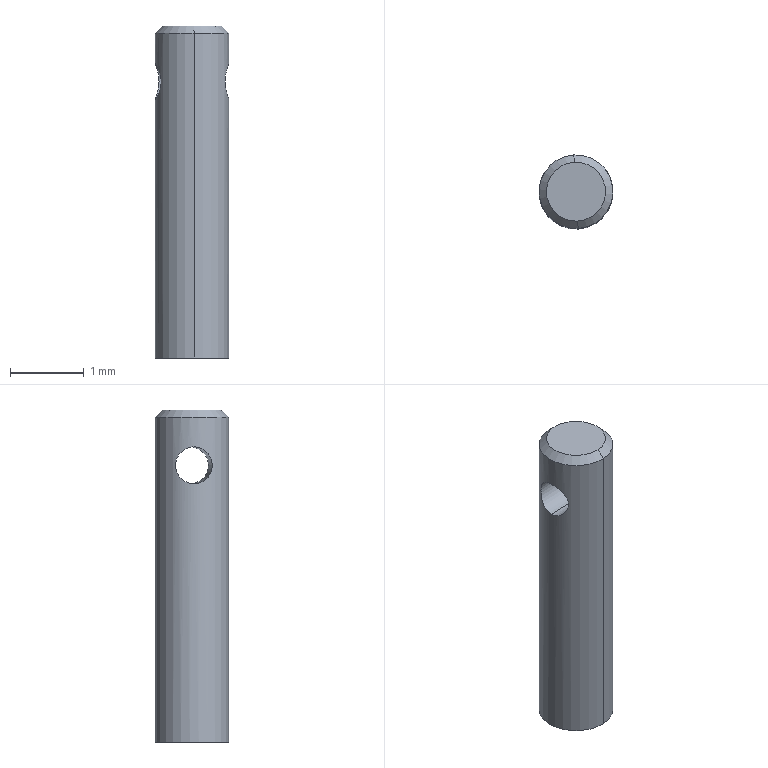Component | SolidWorks | Part25^Assembly1-2 | 1 solid | 8 faces | box 1 x 1 x 4.5 mm | volume 3 mm3 | cylinder 4 | cone 2 | plane 2 | commonest cylinder face diameters 0.5 x2 1 x2
STEP:
#1=COLOUR_RGB('',0.7922,0.8196,0.9333);
#2=FILL_AREA_STYLE_COLOUR('',#1);
#3=FILL_AREA_STYLE('',(#2));
#4=SURFACE_STYLE_FILL_AREA(#3);
#5=SURFACE_SIDE_STYLE('',(#4));
#6=SURFACE_STYLE_USAGE(.BOTH.,#5);
#7=PRESENTATION_STYLE_ASSIGNMENT((#6));
#8=CARTESIAN_POINT('',(0.368,-0.1104,0.3543));
#9=VERTEX_POINT('',#8);
#10=CARTESIAN_POINT('',(0.368,-0.1104,0.3346));
#11=VERTEX_POINT('',#10);
#12=CARTESIAN_POINT('',(0.368,-0.1104,0.3543));
#13=CARTESIAN_POINT('',(0.3682,-0.113,0.3543));
#14=CARTESIAN_POINT('',(0.3689,-0.1156,0.3532));
#15=CARTESIAN_POINT('',(0.3705,-0.1191,0.3496));
#16=CARTESIAN_POINT('',(0.3712,-0.1201,0.3471));
#17=CARTESIAN_POINT('',(0.3712,-0.1201,0.3419));
#18=CARTESIAN_POINT('',(0.3705,-0.1191,0.3393));
#19=CARTESIAN_POINT('',(0.3689,-0.1156,0.3357));
#20=CARTESIAN_POINT('',(0.3682,-0.1131,0.3346));
#21=CARTESIAN_POINT('',(0.368,-0.1104,0.3346));
#22=B_SPLINE_CURVE_WITH_KNOTS('',3,(#12,#13,#14,#15,#16,#17,#18,#19,#20,#21),.UNSPECIFIED.,.F.,.F.,(4,2,2,2,4),(0.0007952,0.0009937,0.001192,0.001391,0.001589),.UNSPECIFIED.);
#23=EDGE_CURVE('',#9,#11,#22,.T.);
#24=ORIENTED_EDGE('',*,*,#23,.F.);
#25=CARTESIAN_POINT('',(0.4073,-0.1082,0.3543));
#26=VERTEX_POINT('',#25);
#27=CARTESIAN_POINT('',(0.4073,-0.1082,0.3543));
#28=DIRECTION('',(0.9983,0.05769,-0.));
#29=VECTOR('',#28,39.37);
#30=LINE('',#27,#29);
#31=EDGE_CURVE('',#9,#26,#30,.T.);
#32=ORIENTED_EDGE('',*,*,#31,.T.);
#33=CARTESIAN_POINT('',(0.4073,-0.1082,0.3346));
#34=VERTEX_POINT('',#33);
#35=CARTESIAN_POINT('',(0.4073,-0.1082,0.3346));
#36=CARTESIAN_POINT('',(0.4075,-0.1108,0.3346));
#37=CARTESIAN_POINT('',(0.407,-0.1134,0.3357));
#38=CARTESIAN_POINT('',(0.4059,-0.117,0.3393));
#39=CARTESIAN_POINT('',(0.4053,-0.1181,0.3419));
#40=CARTESIAN_POINT('',(0.4053,-0.1181,0.3471));
#41=CARTESIAN_POINT('',(0.4059,-0.117,0.3497));
#42=CARTESIAN_POINT('',(0.407,-0.1134,0.3532));
#43=CARTESIAN_POINT('',(0.4075,-0.1108,0.3543));
#44=CARTESIAN_POINT('',(0.4073,-0.1082,0.3543));
#45=B_SPLINE_CURVE_WITH_KNOTS('',3,(#35,#36,#37,#38,#39,#40,#41,#42,#43,#44),.UNSPECIFIED.,.F.,.F.,(4,2,2,2,4),(0.,0.0001988,0.0003976,0.0005964,0.0007952),.UNSPECIFIED.);
#46=EDGE_CURVE('',#34,#26,#45,.T.);
#47=ORIENTED_EDGE('',*,*,#46,.F.);
#48=CARTESIAN_POINT('',(0.4073,-0.1082,0.3346));
#49=DIRECTION('',(0.9983,0.05769,-0.));
#50=VECTOR('',#49,39.37);
#51=LINE('',#48,#50);
#52=EDGE_CURVE('',#11,#34,#51,.T.);
#53=ORIENTED_EDGE('',*,*,#52,.F.);
#54=EDGE_LOOP('',(#24,#32,#47,#53));
#55=FACE_OUTER_BOUND('',#54,.T.);
#56=CARTESIAN_POINT('',(0.4073,-0.1082,0.3445));
#57=DIRECTION('',(0.9983,0.05769,-0.));
#58=DIRECTION('',(0.,0.,-1.));
#59=AXIS2_PLACEMENT_3D('',#56,#57,#58);
#60=CYLINDRICAL_SURFACE('',#59,0.009843);
#61=ADVANCED_FACE('',(#55),#60,.F.);
#62=CARTESIAN_POINT('',(0.3868,-0.09358,0.374));
#63=VERTEX_POINT('',#62);
#64=CARTESIAN_POINT('',(0.3886,-0.125,0.374));
#65=VERTEX_POINT('',#64);
#66=CARTESIAN_POINT('',(0.3877,-0.1093,0.374));
#67=DIRECTION('',(0.,0.,1.));
#68=DIRECTION('',(-0.05769,0.9983,0.));
#69=AXIS2_PLACEMENT_3D('',#66,#67,#68);
#70=CIRCLE('',#69,0.01575);
#71=EDGE_CURVE('',#63,#65,#70,.T.);
#72=ORIENTED_EDGE('',*,*,#71,.F.);
#73=CARTESIAN_POINT('',(0.3865,-0.08965,0.3701));
#74=VERTEX_POINT('',#73);
#75=CARTESIAN_POINT('',(0.3868,-0.09358,0.374));
#76=DIRECTION('',(-0.04079,0.7059,-0.7071));
#77=VECTOR('',#76,39.37);
#78=LINE('',#75,#77);
#79=EDGE_CURVE('',#63,#74,#78,.T.);
#80=ORIENTED_EDGE('',*,*,#79,.T.);
#81=CARTESIAN_POINT('',(0.3888,-0.129,0.3701));
#82=VERTEX_POINT('',#81);
#83=CARTESIAN_POINT('',(0.3877,-0.1093,0.3701));
#84=DIRECTION('',(-0.,-0.,-1.));
#85=DIRECTION('',(-0.05769,0.9983,0.));
#86=AXIS2_PLACEMENT_3D('',#83,#84,#85);
#87=CIRCLE('',#86,0.01969);
#88=EDGE_CURVE('',#82,#74,#87,.T.);
#89=ORIENTED_EDGE('',*,*,#88,.F.);
#90=CARTESIAN_POINT('',(0.3886,-0.125,0.374));
#91=DIRECTION('',(0.04079,-0.7059,-0.7071));
#92=VECTOR('',#91,39.37);
#93=LINE('',#90,#92);
#94=EDGE_CURVE('',#65,#82,#93,.T.);
#95=ORIENTED_EDGE('',*,*,#94,.F.);
#96=EDGE_LOOP('',(#72,#80,#89,#95));
#97=FACE_OUTER_BOUND('',#96,.T.);
#98=CARTESIAN_POINT('',(0.3877,-0.1093,0.374));
#99=DIRECTION('',(-0.,-0.,-1.));
#100=DIRECTION('',(0.05769,-0.9983,0.));
#101=AXIS2_PLACEMENT_3D('',#98,#99,#100);
#102=CONICAL_SURFACE('',#101,0.01575,0.7854);
#103=ADVANCED_FACE('',(#97),#102,.T.);
#104=CARTESIAN_POINT('',(0.368,-0.1104,0.3346));
#105=CARTESIAN_POINT('',(0.3679,-0.1078,0.3346));
#106=CARTESIAN_POINT('',(0.3683,-0.1052,0.3357));
#107=CARTESIAN_POINT('',(0.3695,-0.1016,0.3393));
#108=CARTESIAN_POINT('',(0.3701,-0.1005,0.3419));
#109=CARTESIAN_POINT('',(0.3701,-0.1005,0.3471));
#110=CARTESIAN_POINT('',(0.3695,-0.1016,0.3497));
#111=CARTESIAN_POINT('',(0.3683,-0.1052,0.3532));
#112=CARTESIAN_POINT('',(0.3679,-0.1078,0.3543));
#113=CARTESIAN_POINT('',(0.368,-0.1104,0.3543));
#114=B_SPLINE_CURVE_WITH_KNOTS('',3,(#104,#105,#106,#107,#108,#109,#110,#111,#112,#113),.UNSPECIFIED.,.F.,.F.,(4,2,2,2,4),(0.,0.0001988,0.0003976,0.0005964,0.0007952),.UNSPECIFIED.);
#115=EDGE_CURVE('',#11,#9,#114,.T.);
#116=ORIENTED_EDGE('',*,*,#115,.T.);
#117=ORIENTED_EDGE('',*,*,#23,.T.);
#118=EDGE_LOOP('',(#116,#117));
#119=FACE_BOUND('',#118,.T.);
#120=CARTESIAN_POINT('',(0.3865,-0.08965,0.1969));
#121=VERTEX_POINT('',#120);
#122=CARTESIAN_POINT('',(0.3888,-0.129,0.1969));
#123=VERTEX_POINT('',#122);
#124=CARTESIAN_POINT('',(0.3877,-0.1093,0.1969));
#125=DIRECTION('',(0.,0.,1.));
#126=DIRECTION('',(-0.05769,0.9983,0.));
#127=AXIS2_PLACEMENT_3D('',#124,#125,#126);
#128=CIRCLE('',#127,0.01969);
#129=EDGE_CURVE('',#121,#123,#128,.T.);
#130=ORIENTED_EDGE('',*,*,#129,.T.);
#131=CARTESIAN_POINT('',(0.3888,-0.129,0.1969));
#132=DIRECTION('',(0.,0.,1.));
#133=VECTOR('',#132,39.37);
#134=LINE('',#131,#133);
#135=EDGE_CURVE('',#123,#82,#134,.T.);
#136=ORIENTED_EDGE('',*,*,#135,.T.);
#137=ORIENTED_EDGE('',*,*,#88,.T.);
#138=CARTESIAN_POINT('',(0.3865,-0.08965,0.1969));
#139=DIRECTION('',(0.,0.,1.));
#140=VECTOR('',#139,39.37);
#141=LINE('',#138,#140);
#142=EDGE_CURVE('',#121,#74,#141,.T.);
#143=ORIENTED_EDGE('',*,*,#142,.F.);
#144=EDGE_LOOP('',(#130,#136,#137,#143));
#145=FACE_OUTER_BOUND('',#144,.T.);
#146=CARTESIAN_POINT('',(0.3877,-0.1093,0.1969));
#147=DIRECTION('',(0.,0.,1.));
#148=DIRECTION('',(-0.05769,0.9983,0.));
#149=AXIS2_PLACEMENT_3D('',#146,#147,#148);
#150=CYLINDRICAL_SURFACE('',#149,0.01969);
#151=ADVANCED_FACE('',(#119,#145),#150,.T.);
#152=ORIENTED_EDGE('',*,*,#135,.F.);
#153=CARTESIAN_POINT('',(0.3877,-0.1093,0.1969));
#154=DIRECTION('',(0.,0.,1.));
#155=DIRECTION('',(-0.05769,0.9983,0.));
#156=AXIS2_PLACEMENT_3D('',#153,#154,#155);
#157=CIRCLE('',#156,0.01969);
#158=EDGE_CURVE('',#123,#121,#157,.T.);
#159=ORIENTED_EDGE('',*,*,#158,.T.);
#160=ORIENTED_EDGE('',*,*,#142,.T.);
#161=CARTESIAN_POINT('',(0.3877,-0.1093,0.3701));
#162=DIRECTION('',(-0.,-0.,-1.));
#163=DIRECTION('',(-0.05769,0.9983,0.));
#164=AXIS2_PLACEMENT_3D('',#161,#162,#163);
#165=CIRCLE('',#164,0.01969);
#166=EDGE_CURVE('',#74,#82,#165,.T.);
#167=ORIENTED_EDGE('',*,*,#166,.T.);
#168=EDGE_LOOP('',(#152,#159,#160,#167));
#169=FACE_OUTER_BOUND('',#168,.T.);
#170=ORIENTED_EDGE('',*,*,#46,.T.);
#171=CARTESIAN_POINT('',(0.4073,-0.1082,0.3543));
#172=CARTESIAN_POINT('',(0.4072,-0.1056,0.3543));
#173=CARTESIAN_POINT('',(0.4064,-0.103,0.3532));
#174=CARTESIAN_POINT('',(0.4049,-0.09954,0.3496));
#175=CARTESIAN_POINT('',(0.4041,-0.0985,0.3471));
#176=CARTESIAN_POINT('',(0.4041,-0.09849,0.3419));
#177=CARTESIAN_POINT('',(0.4049,-0.09953,0.3393));
#178=CARTESIAN_POINT('',(0.4064,-0.103,0.3357));
#179=CARTESIAN_POINT('',(0.4072,-0.1055,0.3346));
#180=CARTESIAN_POINT('',(0.4073,-0.1082,0.3346));
#181=B_SPLINE_CURVE_WITH_KNOTS('',3,(#171,#172,#173,#174,#175,#176,#177,#178,#179,#180),.UNSPECIFIED.,.F.,.F.,(4,2,2,2,4),(0.0007952,0.0009937,0.001192,0.001391,0.001589),.UNSPECIFIED.);
#182=EDGE_CURVE('',#26,#34,#181,.T.);
#183=ORIENTED_EDGE('',*,*,#182,.T.);
#184=EDGE_LOOP('',(#170,#183));
#185=FACE_BOUND('',#184,.T.);
#186=CARTESIAN_POINT('',(0.3877,-0.1093,0.1969));
#187=DIRECTION('',(0.,0.,1.));
#188=DIRECTION('',(-0.05769,0.9983,0.));
#189=AXIS2_PLACEMENT_3D('',#186,#187,#188);
#190=CYLINDRICAL_SURFACE('',#189,0.01969);
#191=ADVANCED_FACE('',(#169,#185),#190,.T.);
#192=ORIENTED_EDGE('',*,*,#129,.F.);
#193=ORIENTED_EDGE('',*,*,#158,.F.);
#194=EDGE_LOOP('',(#192,#193));
#195=FACE_OUTER_BOUND('',#194,.T.);
#196=CARTESIAN_POINT('',(0.3877,-0.1093,0.1969));
#197=DIRECTION('',(0.,0.,1.));
#198=DIRECTION('',(-0.05769,0.9983,0.));
#199=AXIS2_PLACEMENT_3D('',#196,#197,#198);
#200=PLANE('',#199);
#201=ADVANCED_FACE('',(#195),#200,.F.);
#202=CARTESIAN_POINT('',(0.3877,-0.1093,0.374));
#203=DIRECTION('',(0.,0.,1.));
#204=DIRECTION('',(-0.05769,0.9983,0.));
#205=AXIS2_PLACEMENT_3D('',#202,#203,#204);
#206=CIRCLE('',#205,0.01575);
#207=EDGE_CURVE('',#65,#63,#206,.T.);
#208=ORIENTED_EDGE('',*,*,#207,.T.);
#209=ORIENTED_EDGE('',*,*,#71,.T.);
#210=EDGE_LOOP('',(#208,#209));
#211=FACE_OUTER_BOUND('',#210,.T.);
#212=CARTESIAN_POINT('',(0.3877,-0.1093,0.374));
#213=DIRECTION('',(0.,0.,1.));
#214=DIRECTION('',(-0.05769,0.9983,0.));
#215=AXIS2_PLACEMENT_3D('',#212,#213,#214);
#216=PLANE('',#215);
#217=ADVANCED_FACE('',(#211),#216,.T.);
#218=ORIENTED_EDGE('',*,*,#79,.F.);
#219=ORIENTED_EDGE('',*,*,#207,.F.);
#220=ORIENTED_EDGE('',*,*,#94,.T.);
#221=ORIENTED_EDGE('',*,*,#166,.F.);
#222=EDGE_LOOP('',(#218,#219,#220,#221));
#223=FACE_OUTER_BOUND('',#222,.T.);
#224=CARTESIAN_POINT('',(0.3877,-0.1093,0.374));
#225=DIRECTION('',(-0.,-0.,-1.));
#226=DIRECTION('',(0.05769,-0.9983,0.));
#227=AXIS2_PLACEMENT_3D('',#224,#225,#226);
#228=CONICAL_SURFACE('',#227,0.01575,0.7854);
#229=ADVANCED_FACE('',(#223),#228,.T.);
#230=ORIENTED_EDGE('',*,*,#31,.F.);
#231=ORIENTED_EDGE('',*,*,#115,.F.);
#232=ORIENTED_EDGE('',*,*,#52,.T.);
#233=ORIENTED_EDGE('',*,*,#182,.F.);
#234=EDGE_LOOP('',(#230,#231,#232,#233));
#235=FACE_OUTER_BOUND('',#234,.T.);
#236=CARTESIAN_POINT('',(0.4073,-0.1082,0.3445));
#237=DIRECTION('',(0.9983,0.05769,-0.));
#238=DIRECTION('',(0.,0.,-1.));
#239=AXIS2_PLACEMENT_3D('',#236,#237,#238);
#240=CYLINDRICAL_SURFACE('',#239,0.009843);
#241=ADVANCED_FACE('',(#235),#240,.F.);
#242=CLOSED_SHELL('',(#61,#103,#151,#191,#201,#217,#229,#241));
#243=MANIFOLD_SOLID_BREP('',#242);
#244=STYLED_ITEM('',(#7),#243);
#245=PRESENTATION_LAYER_ASSIGNMENT('','',(#244));
#246=CARTESIAN_POINT('',(0.,0.,0.));
#247=DIRECTION('',(0.,0.,1.));
#248=DIRECTION('',(1.,0.,0.));
#249=AXIS2_PLACEMENT_3D('',#246,#247,#248);
#250=(LENGTH_UNIT()NAMED_UNIT(*)SI_UNIT($,.METRE.));
#251=LENGTH_MEASURE_WITH_UNIT(LENGTH_MEASURE(0.0254),#250);
#252=DIMENSIONAL_EXPONENTS(1.,0.,0.,0.,0.,0.,0.);
#253=(CONVERSION_BASED_UNIT('',#251)LENGTH_UNIT()NAMED_UNIT(#252));
#254=UNCERTAINTY_MEASURE_WITH_UNIT(LENGTH_MEASURE(0.00001),#253,'','');
#255=(NAMED_UNIT(*)PLANE_ANGLE_UNIT()SI_UNIT($,.RADIAN.));
#256=(NAMED_UNIT(*)SI_UNIT($,.STERADIAN.)SOLID_ANGLE_UNIT());
#257=(GEOMETRIC_REPRESENTATION_CONTEXT(3)GLOBAL_UNCERTAINTY_ASSIGNED_CONTEXT((#254))GLOBAL_UNIT_ASSIGNED_CONTEXT((#253,#255,#256))REPRESENTATION_CONTEXT('',''));
#258=ADVANCED_BREP_SHAPE_REPRESENTATION('',(#243,#249),#257);
#259=(LENGTH_UNIT()NAMED_UNIT(*)SI_UNIT($,.METRE.));
#260=LENGTH_MEASURE_WITH_UNIT(LENGTH_MEASURE(0.0254),#259);
#261=DIMENSIONAL_EXPONENTS(1.,0.,0.,0.,0.,0.,0.);
#262=(CONVERSION_BASED_UNIT('',#260)LENGTH_UNIT()NAMED_UNIT(#261));
#263=UNCERTAINTY_MEASURE_WITH_UNIT(LENGTH_MEASURE(0.00001),#262,'','');
#264=(NAMED_UNIT(*)PLANE_ANGLE_UNIT()SI_UNIT($,.RADIAN.));
#265=(NAMED_UNIT(*)SI_UNIT($,.STERADIAN.)SOLID_ANGLE_UNIT());
#266=(GEOMETRIC_REPRESENTATION_CONTEXT(3)GLOBAL_UNCERTAINTY_ASSIGNED_CONTEXT((#263))GLOBAL_UNIT_ASSIGNED_CONTEXT((#262,#264,#265))REPRESENTATION_CONTEXT('',''));
#267=MECHANICAL_DESIGN_GEOMETRIC_PRESENTATION_REPRESENTATION('',(#244),#266);